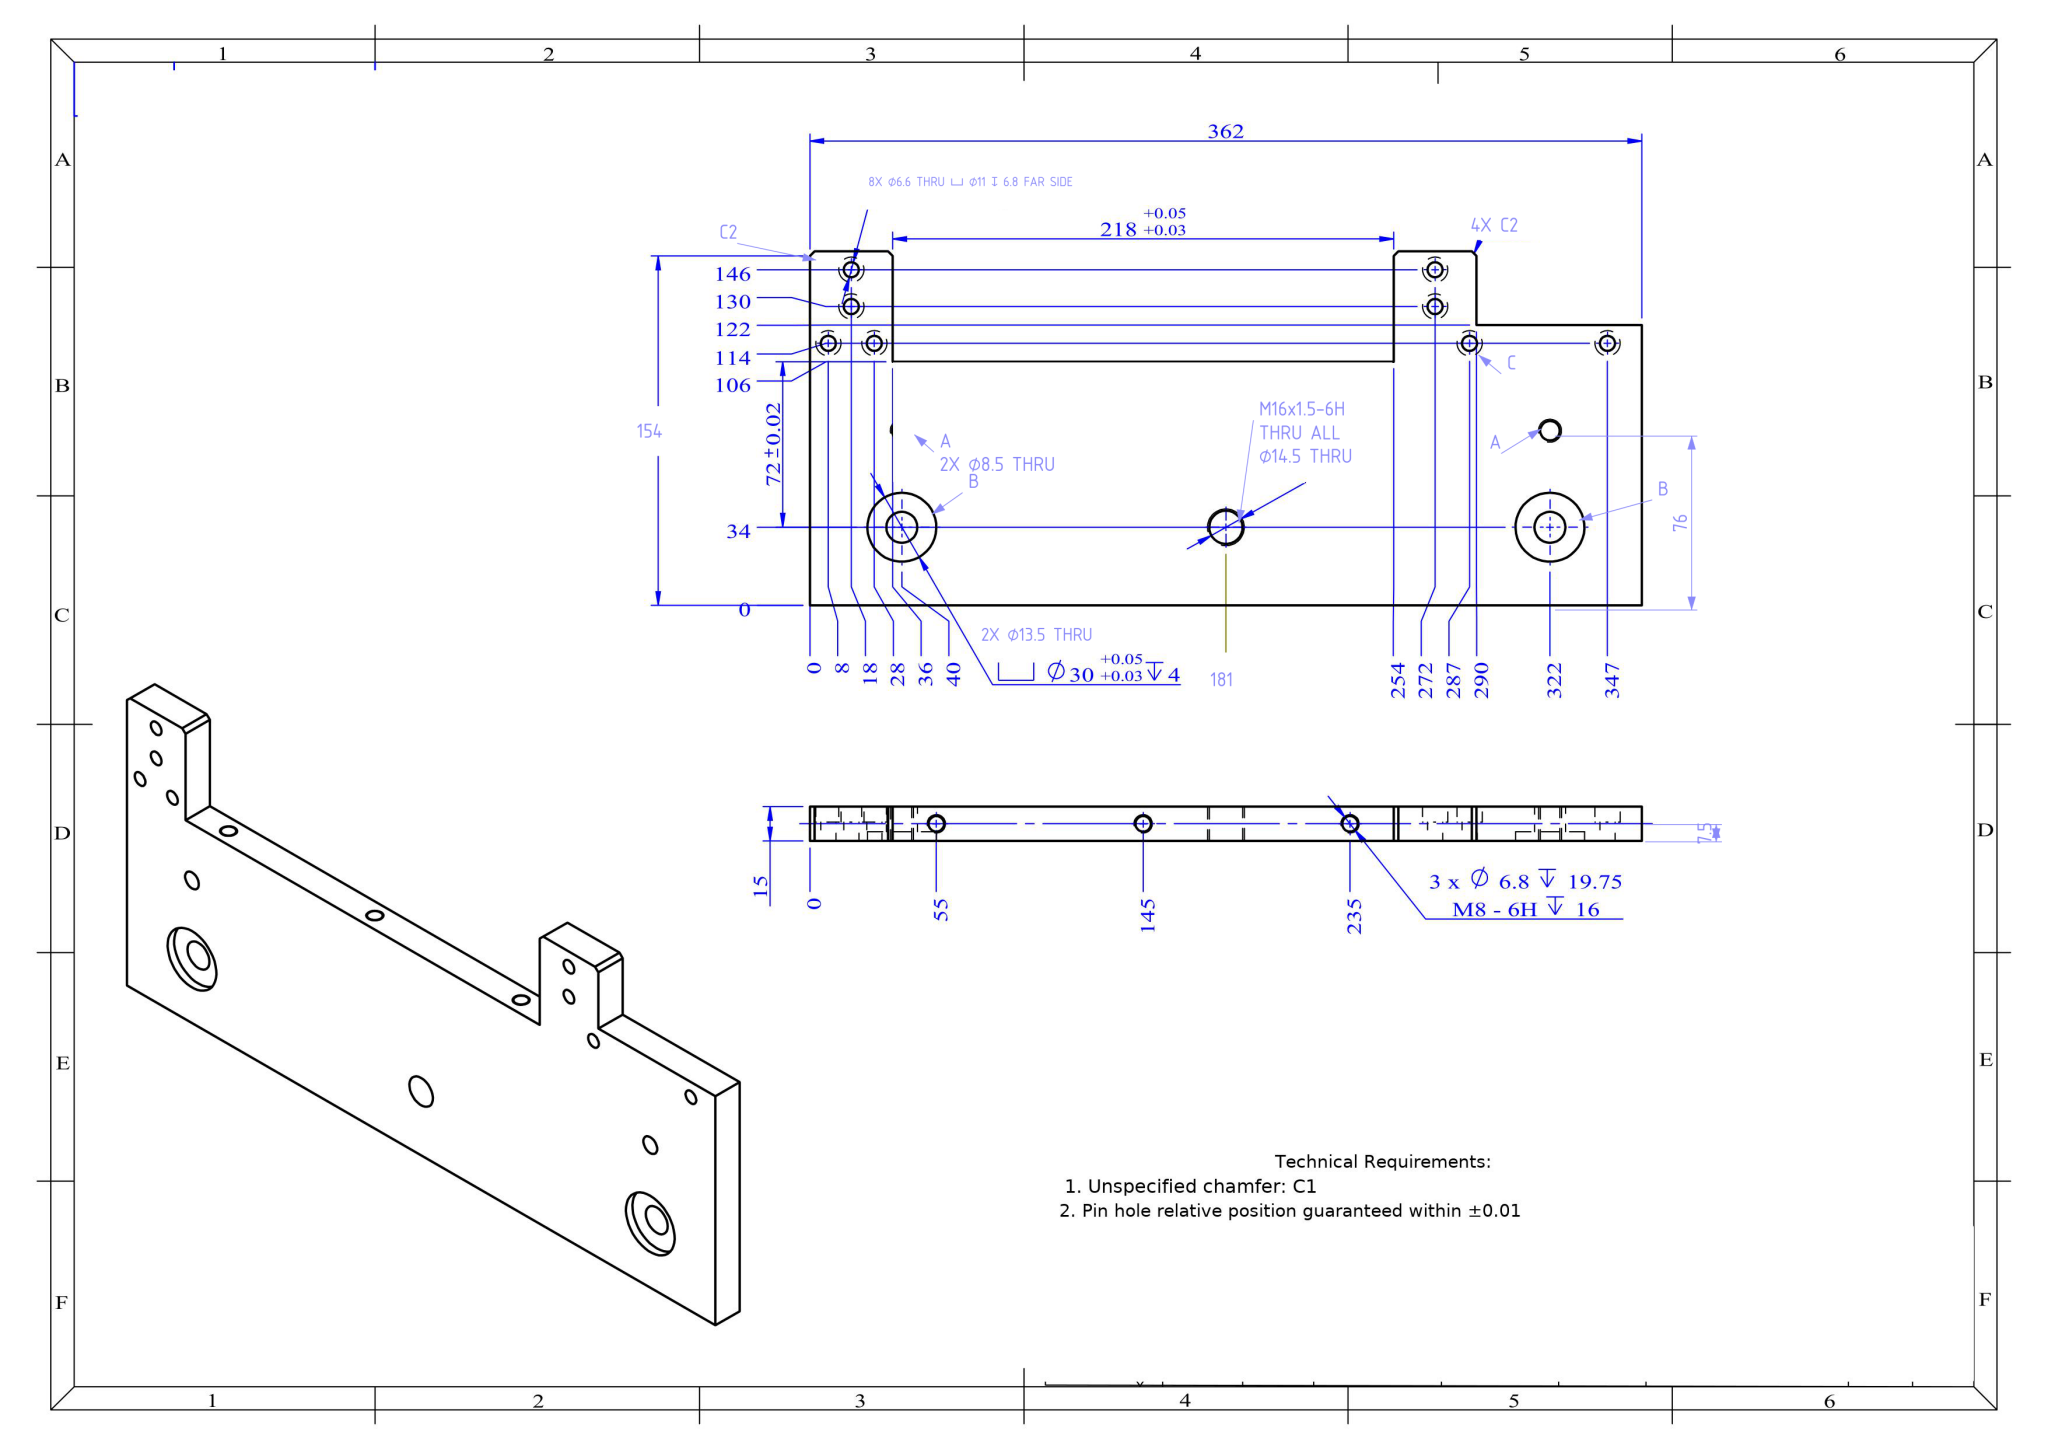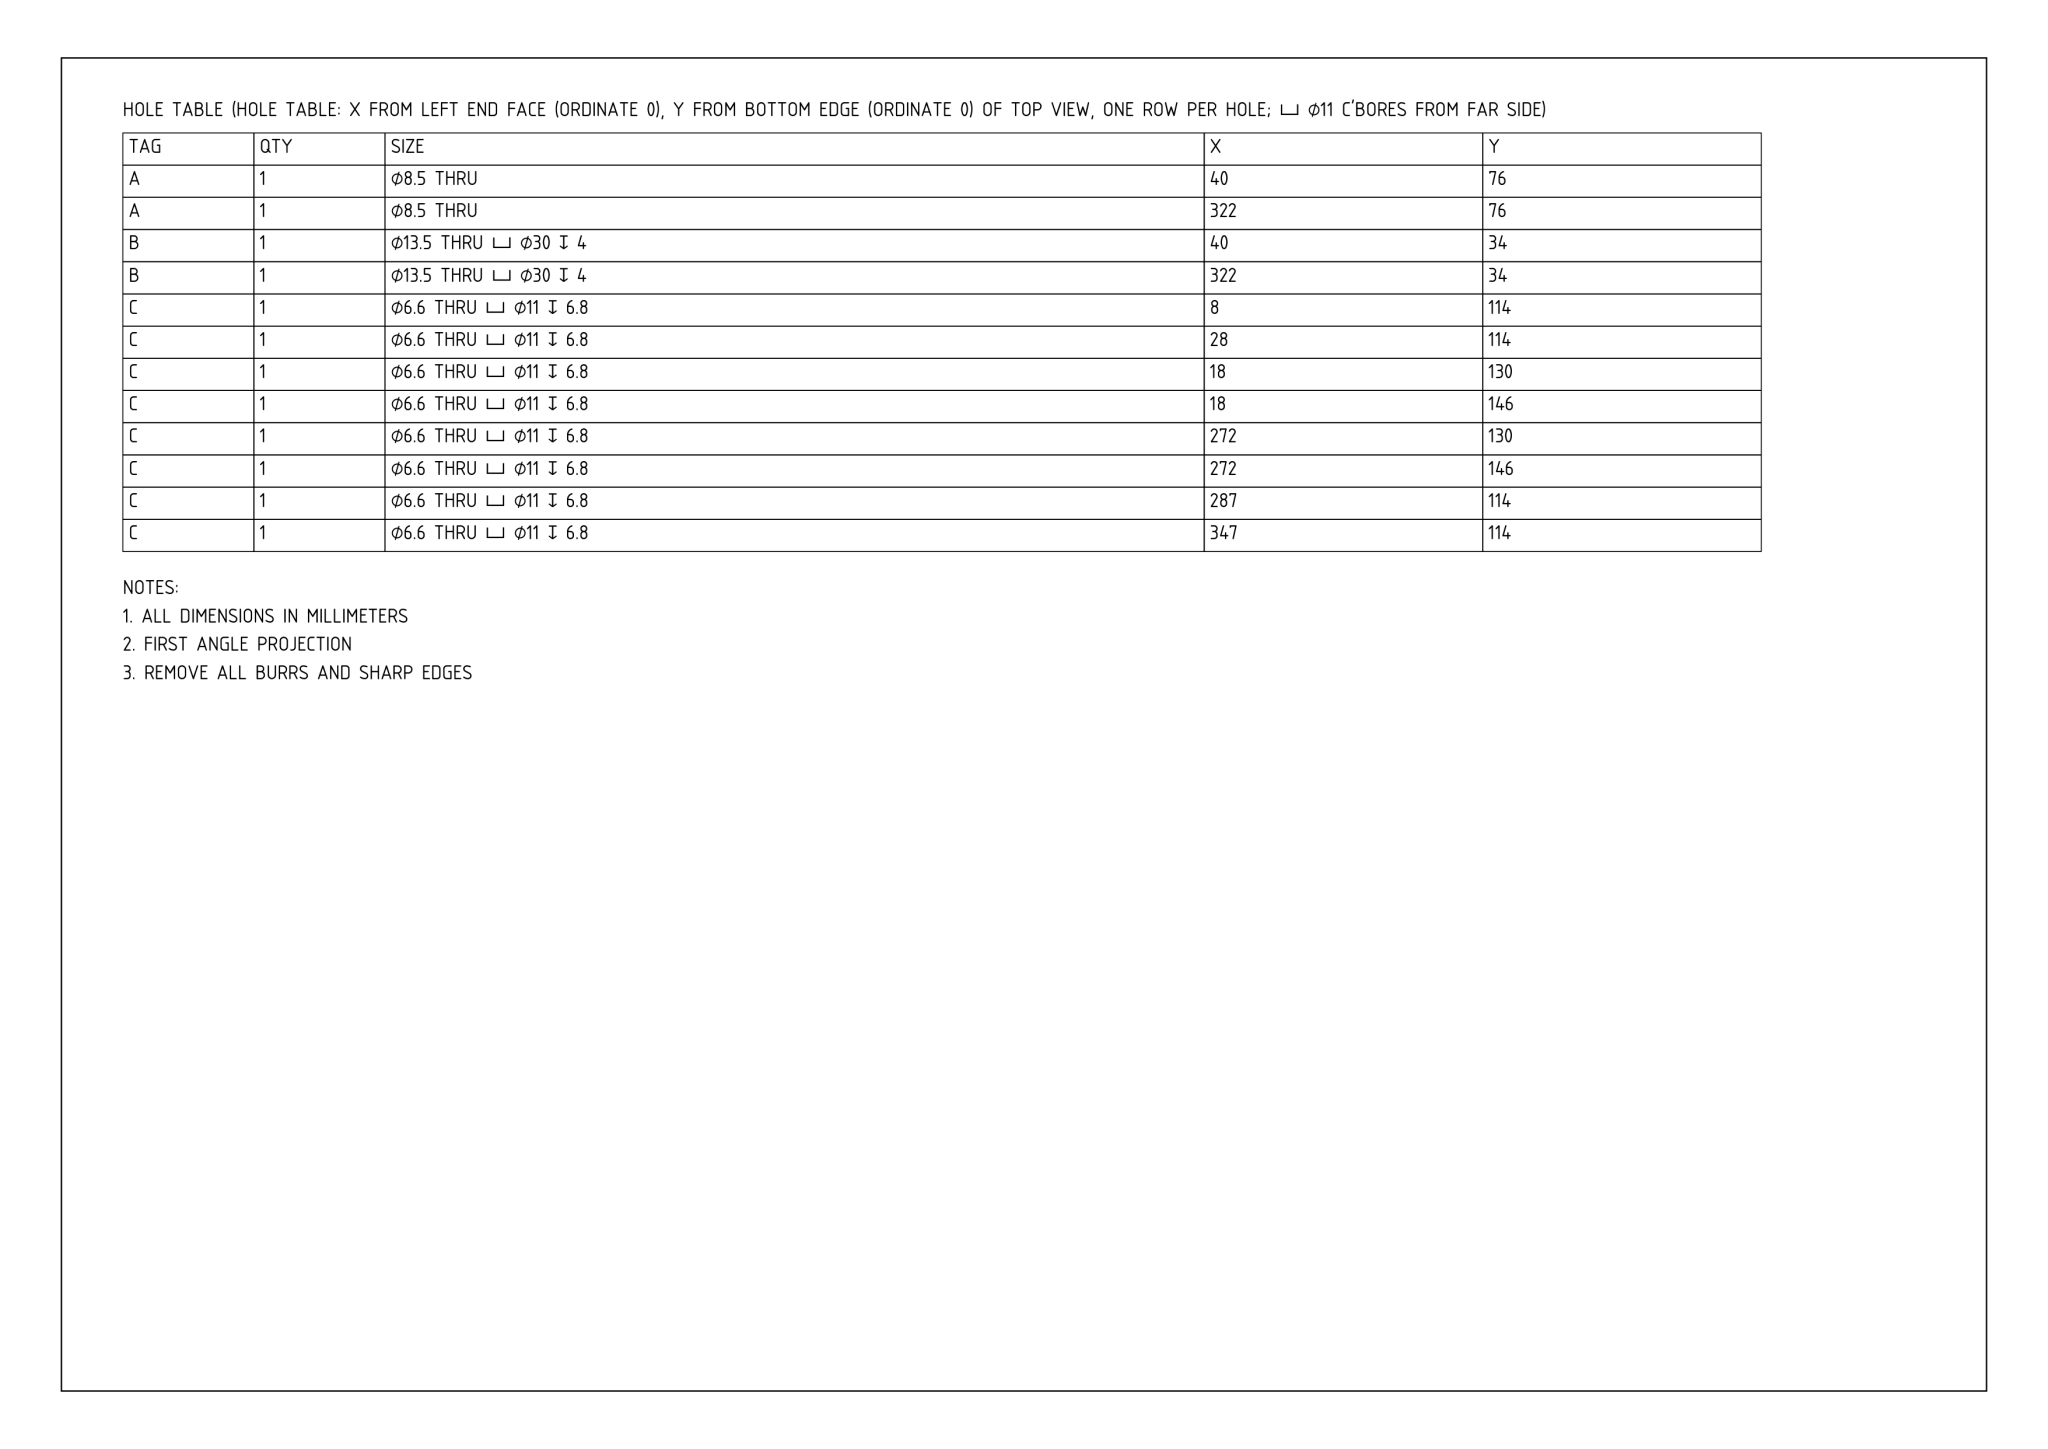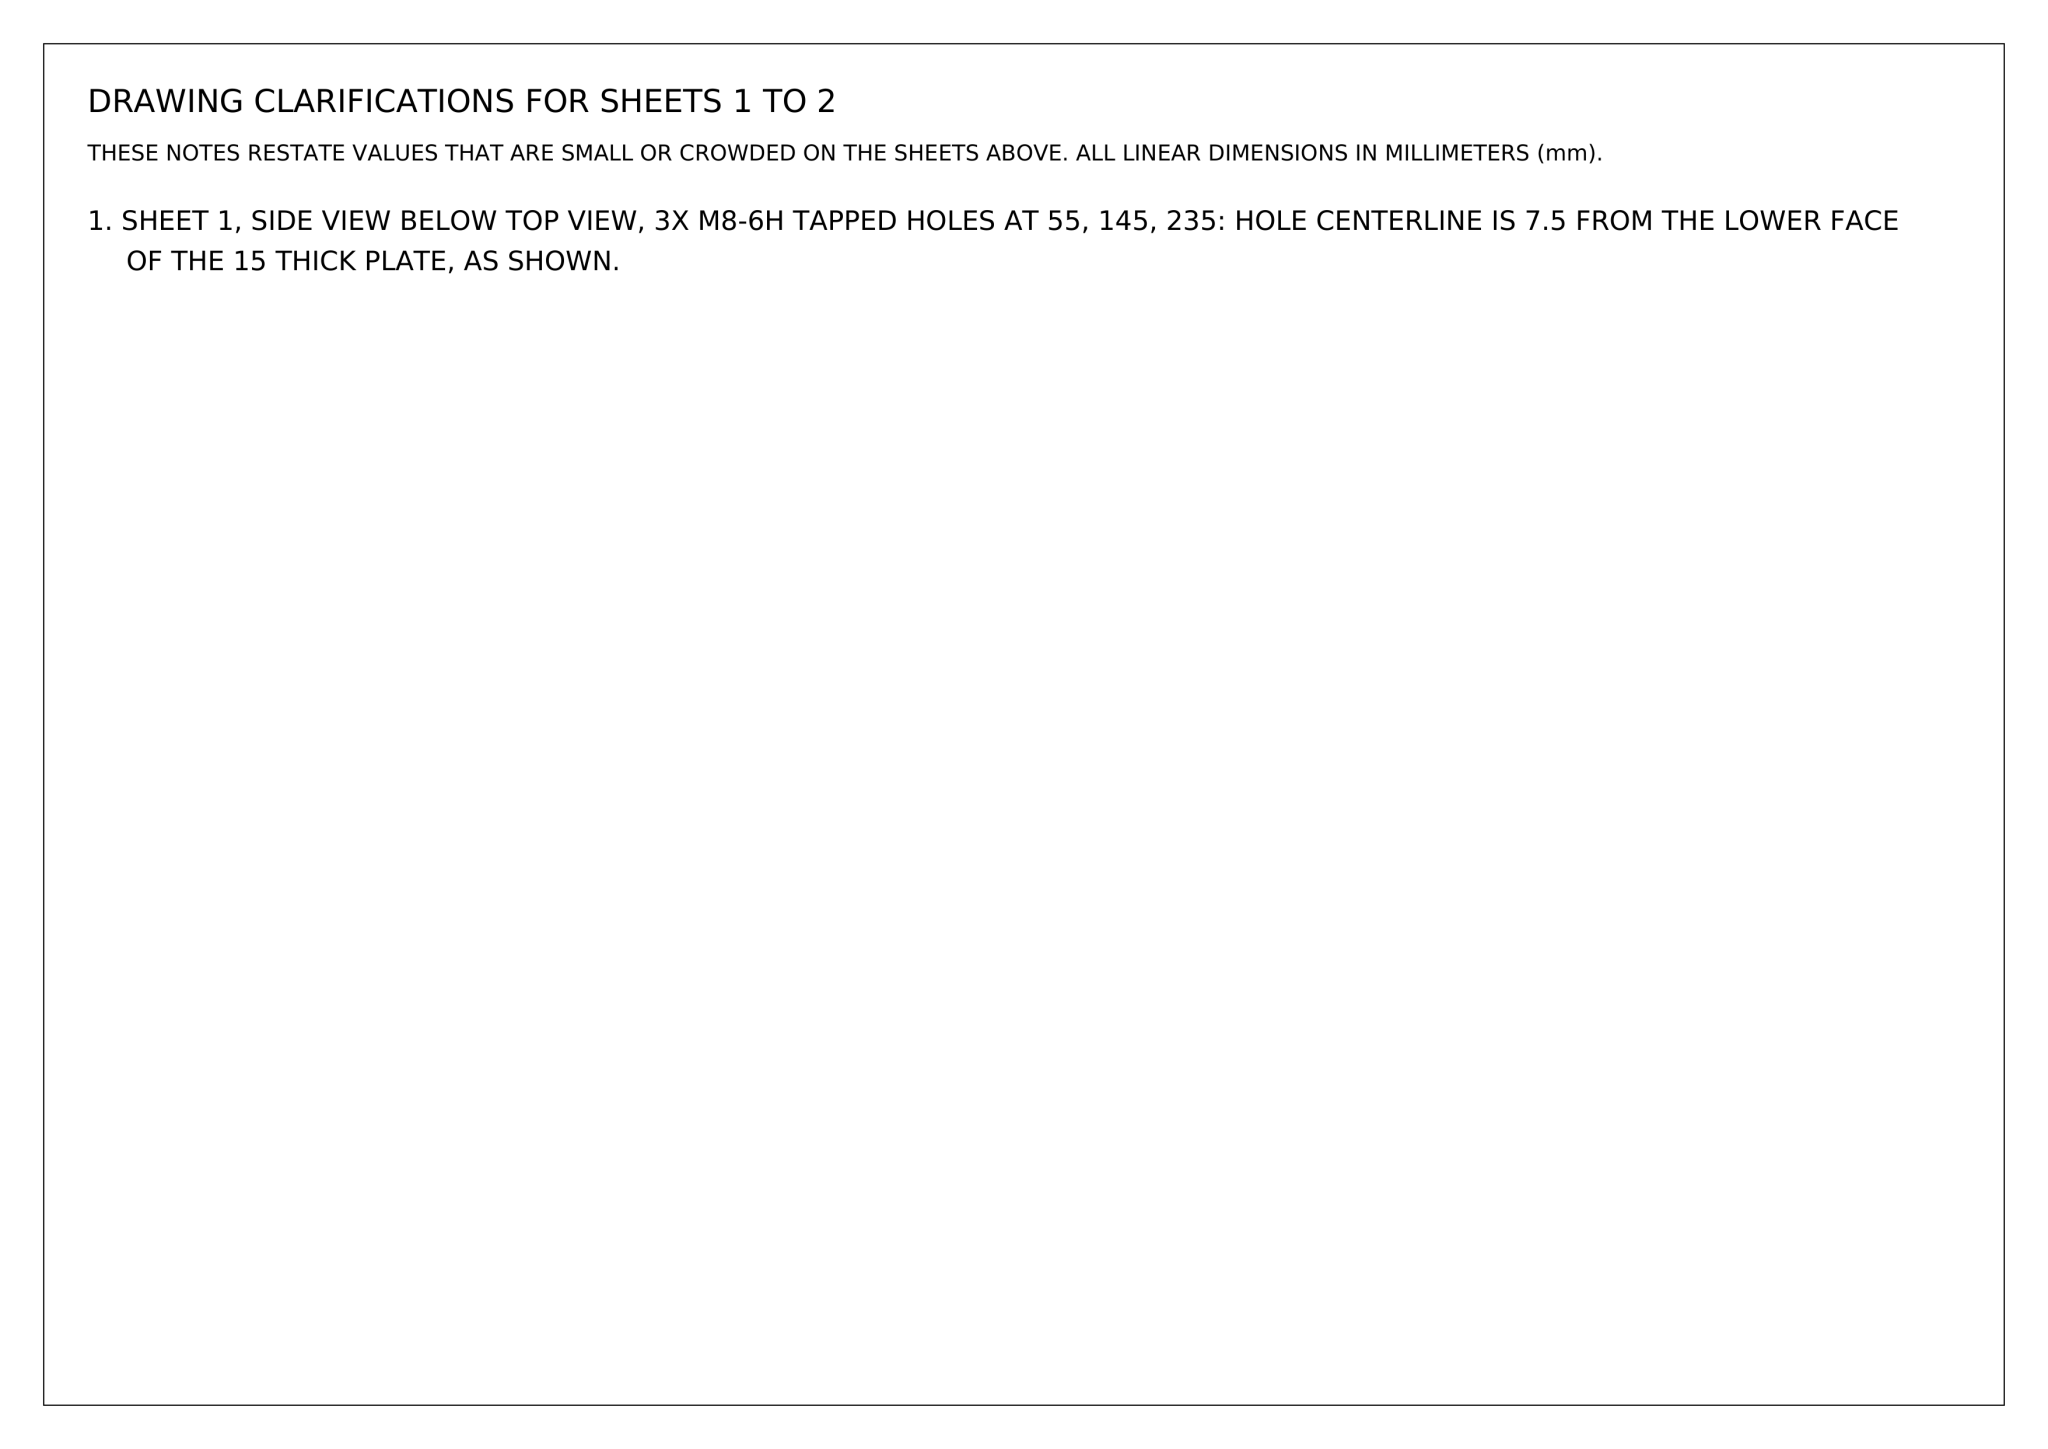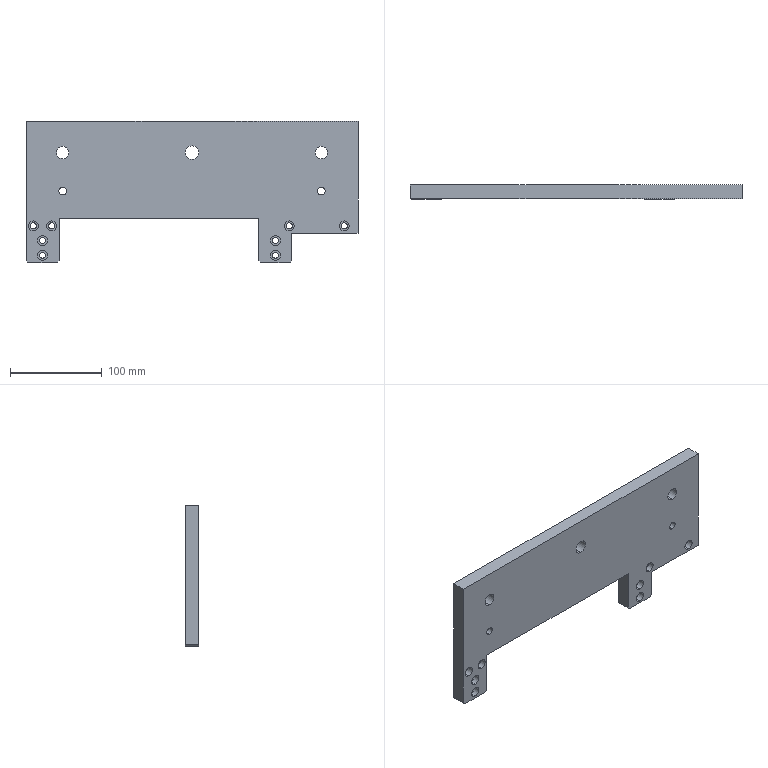Part | NX | mm | 1 solid | 84 faces | box 362 x 15 x 154 mm | volume 621957 mm3 | cylinder 52 | plane 26 | cone 6 | commonest cylinder face diameters 11 x16 6.6 x16 6.8 x6 8.5 x4 13.5 x4 30 x4 14.5 x2